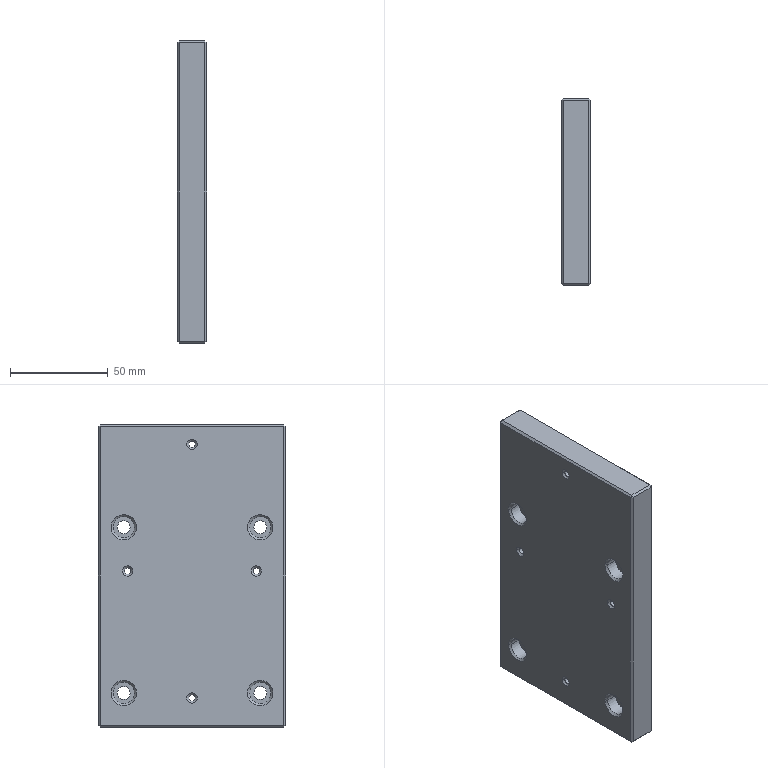Component | SolidWorks | Gasket5-1 | 1 solid | 86 faces | box 15 x 96 x 155 mm | volume 218284 mm3 | cone 32 | plane 30 | cylinder 24 | commonest cylinder face diameters 3.3 x8 11 x8 6.6 x8 | material 1060 Alloy
build123d program:
from build123d import *

# Parameters (mm, degrees)
SKETCH1_W                                          = 96
SKETCH1_H                                          = 155
BOSS_EXTRUDE1_DEPTH                                = 15
HOLE_SIZE_ACCORDING_TO_TYPE_OF_HEXAGON_D           = 6.6
HOLE_SIZE_ACCORDING_TO_TYPE_OF_HEXAGON_CBORE_D     = 11
HOLE_SIZE_ACCORDING_TO_TYPE_OF_HEXAGON_CBORE_DEPTH = 6.8
M4_TAPPED_HOLE1_D                                  = 3.3
CHAMFER1_SIZE                                      = 1


with BuildPart() as part:
    # Sketch1 → Boss-Extrude1 (new body)
    with BuildSketch(Plane.XY):
        Rectangle(SKETCH1_W, SKETCH1_H)
    extrude(amount=BOSS_EXTRUDE1_DEPTH)

    # Hole Size _according to_ type of Hexagon (through all)
    with Locations(Plane.XY.offset(15)):
        with Locations((-35, 60), (35, 60), (35, -25), (-35, -25)):
            CounterBoreHole(HOLE_SIZE_ACCORDING_TO_TYPE_OF_HEXAGON_D / 2, HOLE_SIZE_ACCORDING_TO_TYPE_OF_HEXAGON_CBORE_D / 2, HOLE_SIZE_ACCORDING_TO_TYPE_OF_HEXAGON_CBORE_DEPTH)

    # M4 Tapped Hole1 (through all)
    with Locations(Plane.XY.offset(15)):
        with Locations((0, 62.5), (0, -67.5), (33, -2.5), (-33, -2.5)):
            Hole(M4_TAPPED_HOLE1_D / 2)

    # Chamfer1
    chamfer1_edges = [part.edges().sort_by_distance(p)[0] for p in [
        (48, 0, 15),
        (0, 77.5, 15),
        (-40.5, -25, 15),
        (-31.7, -25, 0),
        (29.5, -25, 15),
        (38.3, -25, 0),
        (29.5, 60, 15),
        (38.3, 60, 0),
        (-40.5, 60, 15),
        (-31.7, 60, 0),
        (-48, 0, 15),
        (0, 77.5, 0),
        (-31.35, -2.5, 15),
        (-31.35, -2.5, 0),
        (48, 0, 0),
        (34.65, -2.5, 15),
        (34.65, -2.5, 0),
        (0, -77.5, 0),
        (-48, 0, 0),
        (1.65, -67.5, 15),
        (1.65, -67.5, 0),
        (1.65, 62.5, 15),
        (1.65, 62.5, 0),
        (0, -77.5, 15),
        (-48, 77.5, 7.5),
        (48, 77.5, 7.5),
        (48, -77.5, 7.5),
        (-48, -77.5, 7.5),
    ]]
    chamfer(chamfer1_edges, length=CHAMFER1_SIZE)


solid = part.part

# Placed as in the assembly
solid = solid.moved(Location((-164.666, 347.264, 248.5), (-90, -90, 0)))